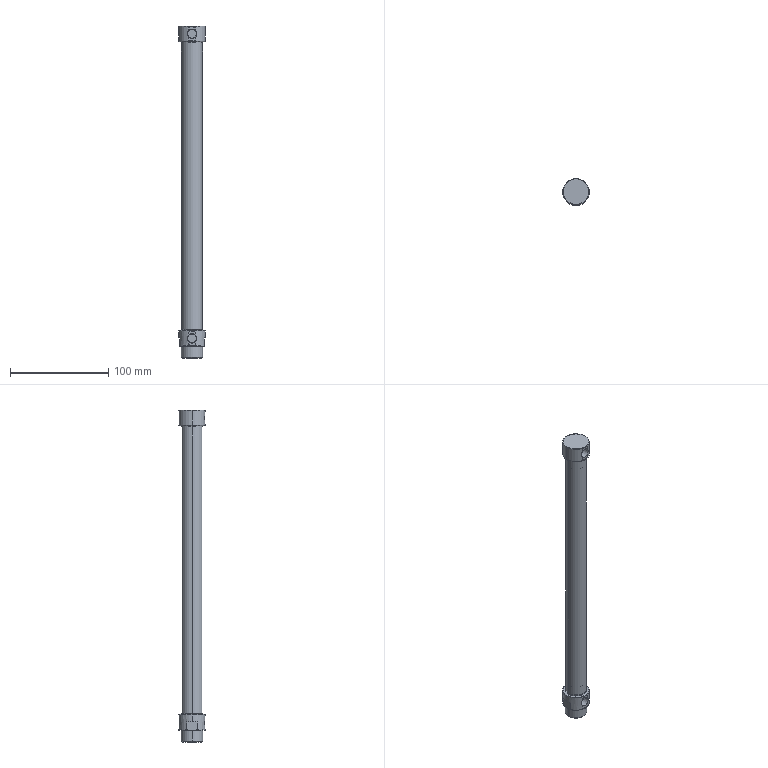Component | SolidWorks | F01AE00111-A2000-21TopEdgeAssembly-1_MA20x250SU(0)+(CS1-M-2)-1_20MAU250 Body-1 | 1 solid | 61 faces | box 27 x 27 x 338 mm | volume 39882 mm3 | cylinder 24 | plane 19 | cone 10 | torus 8 | commonest cylinder face diameters 21.4 x6 9.728 x4 27 x4 14.5 x4 20 x2 8 x2 22 x2
build123d program:
from build123d import *

# Parameters (mm, degrees)
SKETCH2_2_W                 = 37
SKETCH2_2_H                 = 37
SKETCH2_2_W_2               = 25
SKETCH2_2_H_2               = 27
CUT_EXTRUDE1_DEPTH          = 8.5
SKETCH3_R                   = 7.25
IR_PORTSPOTFACE_D14_5_DEPTH = 0.5


with BuildPart() as part:
    # Sketch1_2 → Revolve1 (revolve)
    with BuildSketch(Plane.XY, mode=Mode.PRIVATE) as revolve1_sk:
        with BuildLine():
            Line((0, 0), (0, 10.08))
            Line((0, 10.08), (0.92, 11))
            Line((0.92, 11), (12, 11))
            Line((12, 11), (12, 13.1))
            ThreePointArc((12, 13.1), (12.117, 13.383), (12.4, 13.5))
            Line((12.4, 13.5), (27.6, 13.5))
            ThreePointArc((27.6, 13.5), (27.883, 13.383), (28, 13.1))
            Line((28, 13.1), (28, 10.7))
            Line((28, 10.7), (29, 10.7))
            Line((29, 10.7), (29, 10.2))
            Line((29, 10.2), (29.3, 10.7))
            Line((29.3, 10.7), (320.7, 10.7))
            Line((320.7, 10.7), (321, 10.2))
            Line((321, 10.2), (321, 10.7))
            Line((321, 10.7), (322, 10.7))
            Line((322, 10.7), (322, 13.1))
            ThreePointArc((322, 13.1), (322.117, 13.383), (322.4, 13.5))
            Line((322.4, 13.5), (337.6, 13.5))
            ThreePointArc((337.6, 13.5), (337.883, 13.383), (338, 13.1))
            Line((338, 13.1), (338, 0))
            Line((338, 0), (0, 0))
        make_face()
    revolve(revolve1_sk.sketch.rotate(Axis((338, 0, 0), (-1, 0, 0)), 270), axis=Axis((338, 0, 0), (-1, 0, 0)))

    # Sketch2_2 → Cut-Extrude1 (cut)
    with BuildSketch(Plane(origin=(12, 0, 0), x_dir=(0, 0, -1), z_dir=(1, 0, 0))):
        Rectangle(SKETCH2_2_W, SKETCH2_2_H)
        Rectangle(SKETCH2_2_W_2, SKETCH2_2_H_2, mode=Mode.SUBTRACT)
    extrude(amount=CUT_EXTRUDE1_DEPTH, mode=Mode.SUBTRACT)

    # Sketch3_2 → Cut-Revolve1 (revolve, cut)
    with BuildSketch(Plane.XY, mode=Mode.PRIVATE) as cut_revolve1_sk:
        Polygon((20, 13.5), (24.864, 13.5), (24.283, 12.919), (24.283, 5.5), (20, 5.5), align=None)
    revolve(cut_revolve1_sk.sketch.rotate(Axis((20, 5.5, 0), (0, 1, 0)), 270), axis=Axis((20, 5.5, 0), (0, 1, 0)), mode=Mode.SUBTRACT)

    # Sketch4 → Cut-Revolve2 (revolve, cut)
    with BuildSketch(Plane.XY, mode=Mode.PRIVATE) as cut_revolve2_sk:
        Polygon((330, 13.5), (334.864, 13.5), (334.283, 12.919), (334.283, 5.5), (330, 5.5), align=None)
    revolve(cut_revolve2_sk.sketch.rotate(Axis((330, 5.5, 0), (0, 1, 0)), 270), axis=Axis((330, 5.5, 0), (0, 1, 0)), mode=Mode.SUBTRACT)

    # Sketch5 → Cut-Revolve3 (revolve, cut)
    with BuildSketch(Plane.XY, mode=Mode.PRIVATE) as cut_revolve3_sk:
        Polygon((0, 0), (0, 4), (39, 4), (39, 10), (311, 10), (311, 0), align=None)
    revolve(cut_revolve3_sk.sketch.rotate(Axis((311, 0, 0), (-1, 0, 0)), 270), axis=Axis((311, 0, 0), (-1, 0, 0)), mode=Mode.SUBTRACT)

    # Sketch1 → IR_PortRc18_Major_A (revolve, cut)
    with BuildSketch(Plane.XY, mode=Mode.PRIVATE) as ir_portrc18_major_a_sk:
        Polygon((326.1, 5.5), (325.717, 5.5), (325.136, 6.081), (325.136, 13.9), (326.1, 13.9), align=None)
    revolve(ir_portrc18_major_a_sk.sketch.rotate(Axis((330, 3, 0), (0, 1, 0)), 270), axis=Axis((330, 3, 0), (0, 1, 0)), mode=Mode.SUBTRACT)

    # Sketch2 → IR_PortRc18_Major_B (revolve, cut)
    with BuildSketch(Plane.XY, mode=Mode.PRIVATE) as ir_portrc18_major_b_sk:
        Polygon((16.1, 5.5), (15.717, 5.5), (15.136, 6.081), (15.136, 13.9), (16.1, 13.9), align=None)
    revolve(ir_portrc18_major_b_sk.sketch.rotate(Axis((20, 3, 0), (0, 1, 0)), 270), axis=Axis((20, 3, 0), (0, 1, 0)), mode=Mode.SUBTRACT)

    # Sketch3 → IR_PortSpotFace_D14.5 (cut, symmetric)
    with BuildSketch(Plane(origin=(0, 13.5, 0), x_dir=(1, 0, 0), z_dir=(0, 1, 0))):
        with Locations((330, 0)):
            Circle(SKETCH3_R)
        with Locations((20, 0)):
            Circle(SKETCH3_R)
    extrude(amount=IR_PORTSPOTFACE_D14_5_DEPTH, both=True, mode=Mode.SUBTRACT)


solid = part.part

# Placed as in the assembly
solid = solid.moved(Location((-109.352, 82.548, -343.975), (180, 90, 0)))